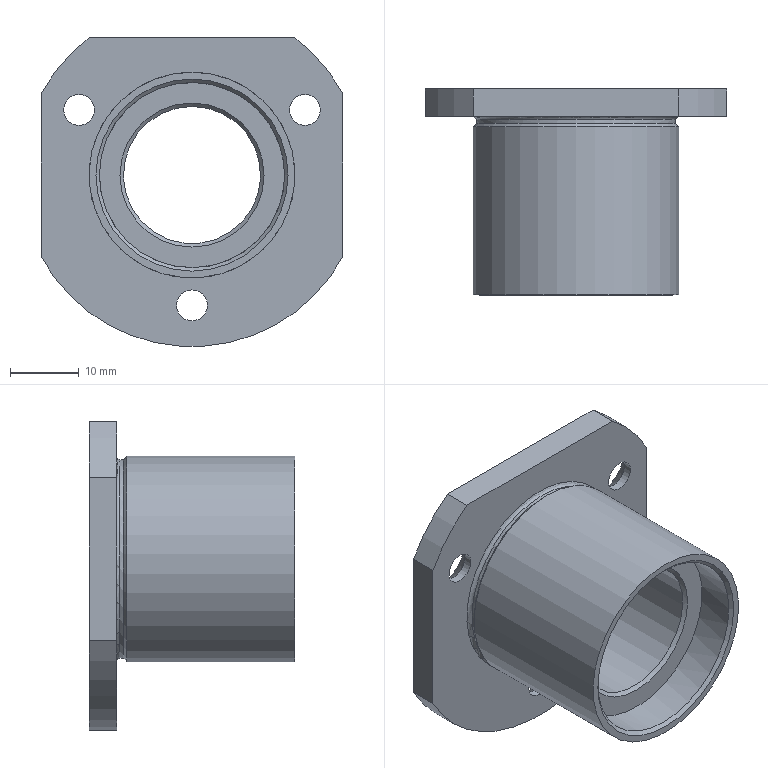Component | NX | INDEXING_SLEEVE | 1 solid | 25 faces | volume 13967 mm3 | cylinder 10 | plane 7 | cone 7 | torus 1 | commonest cylinder face diameters 50 x3 4.5 x3 30 x1 29 x1 27 x1 20 x1